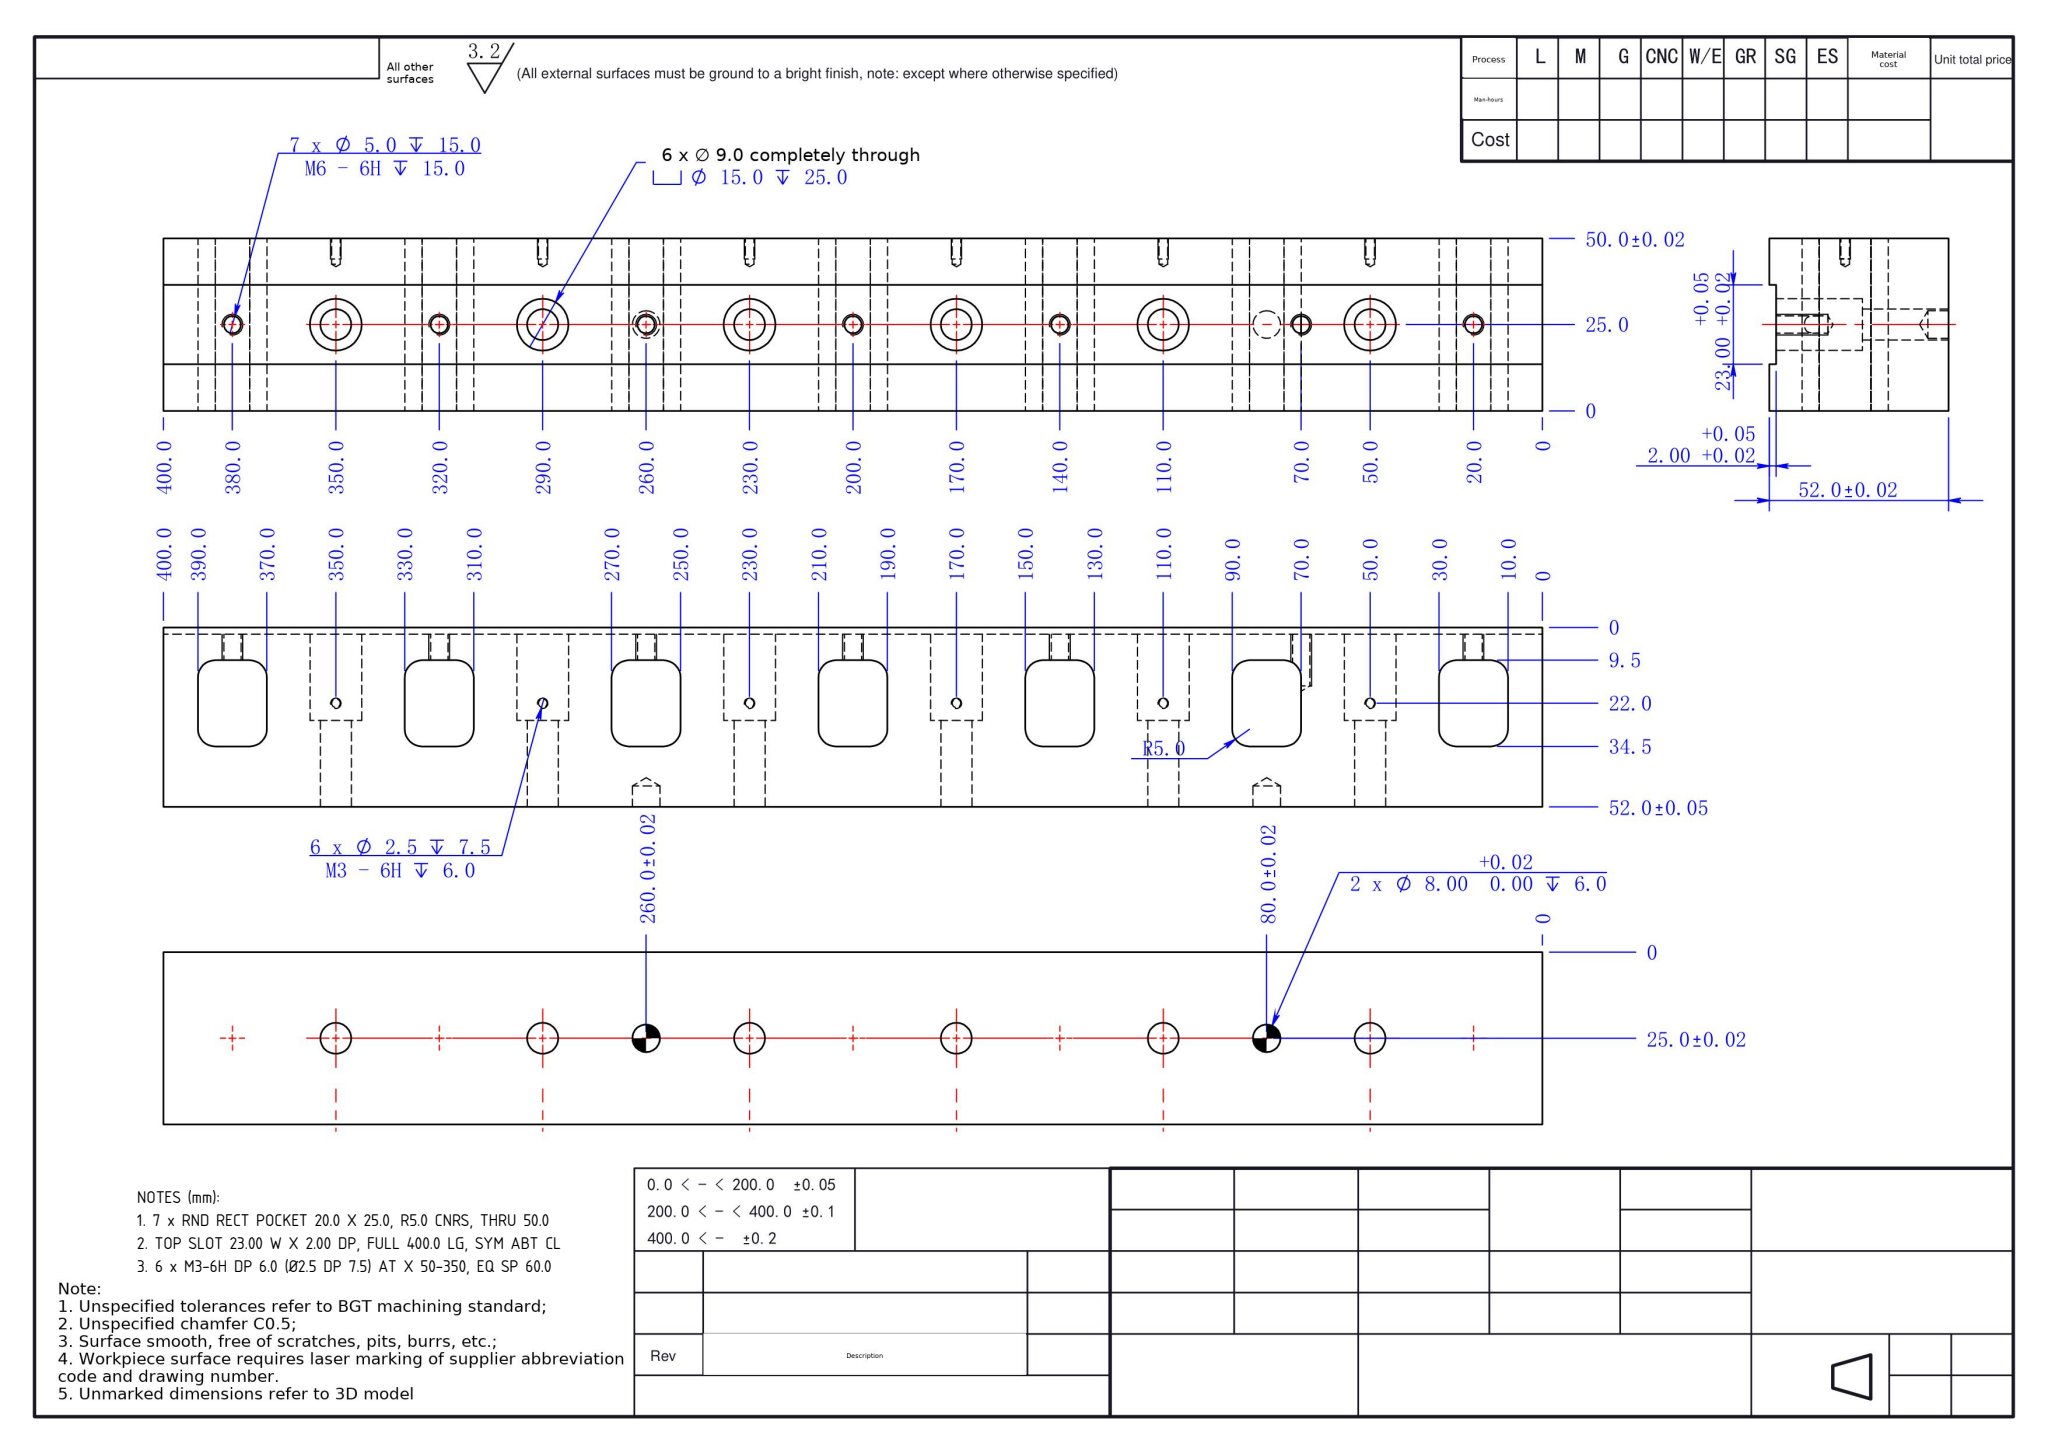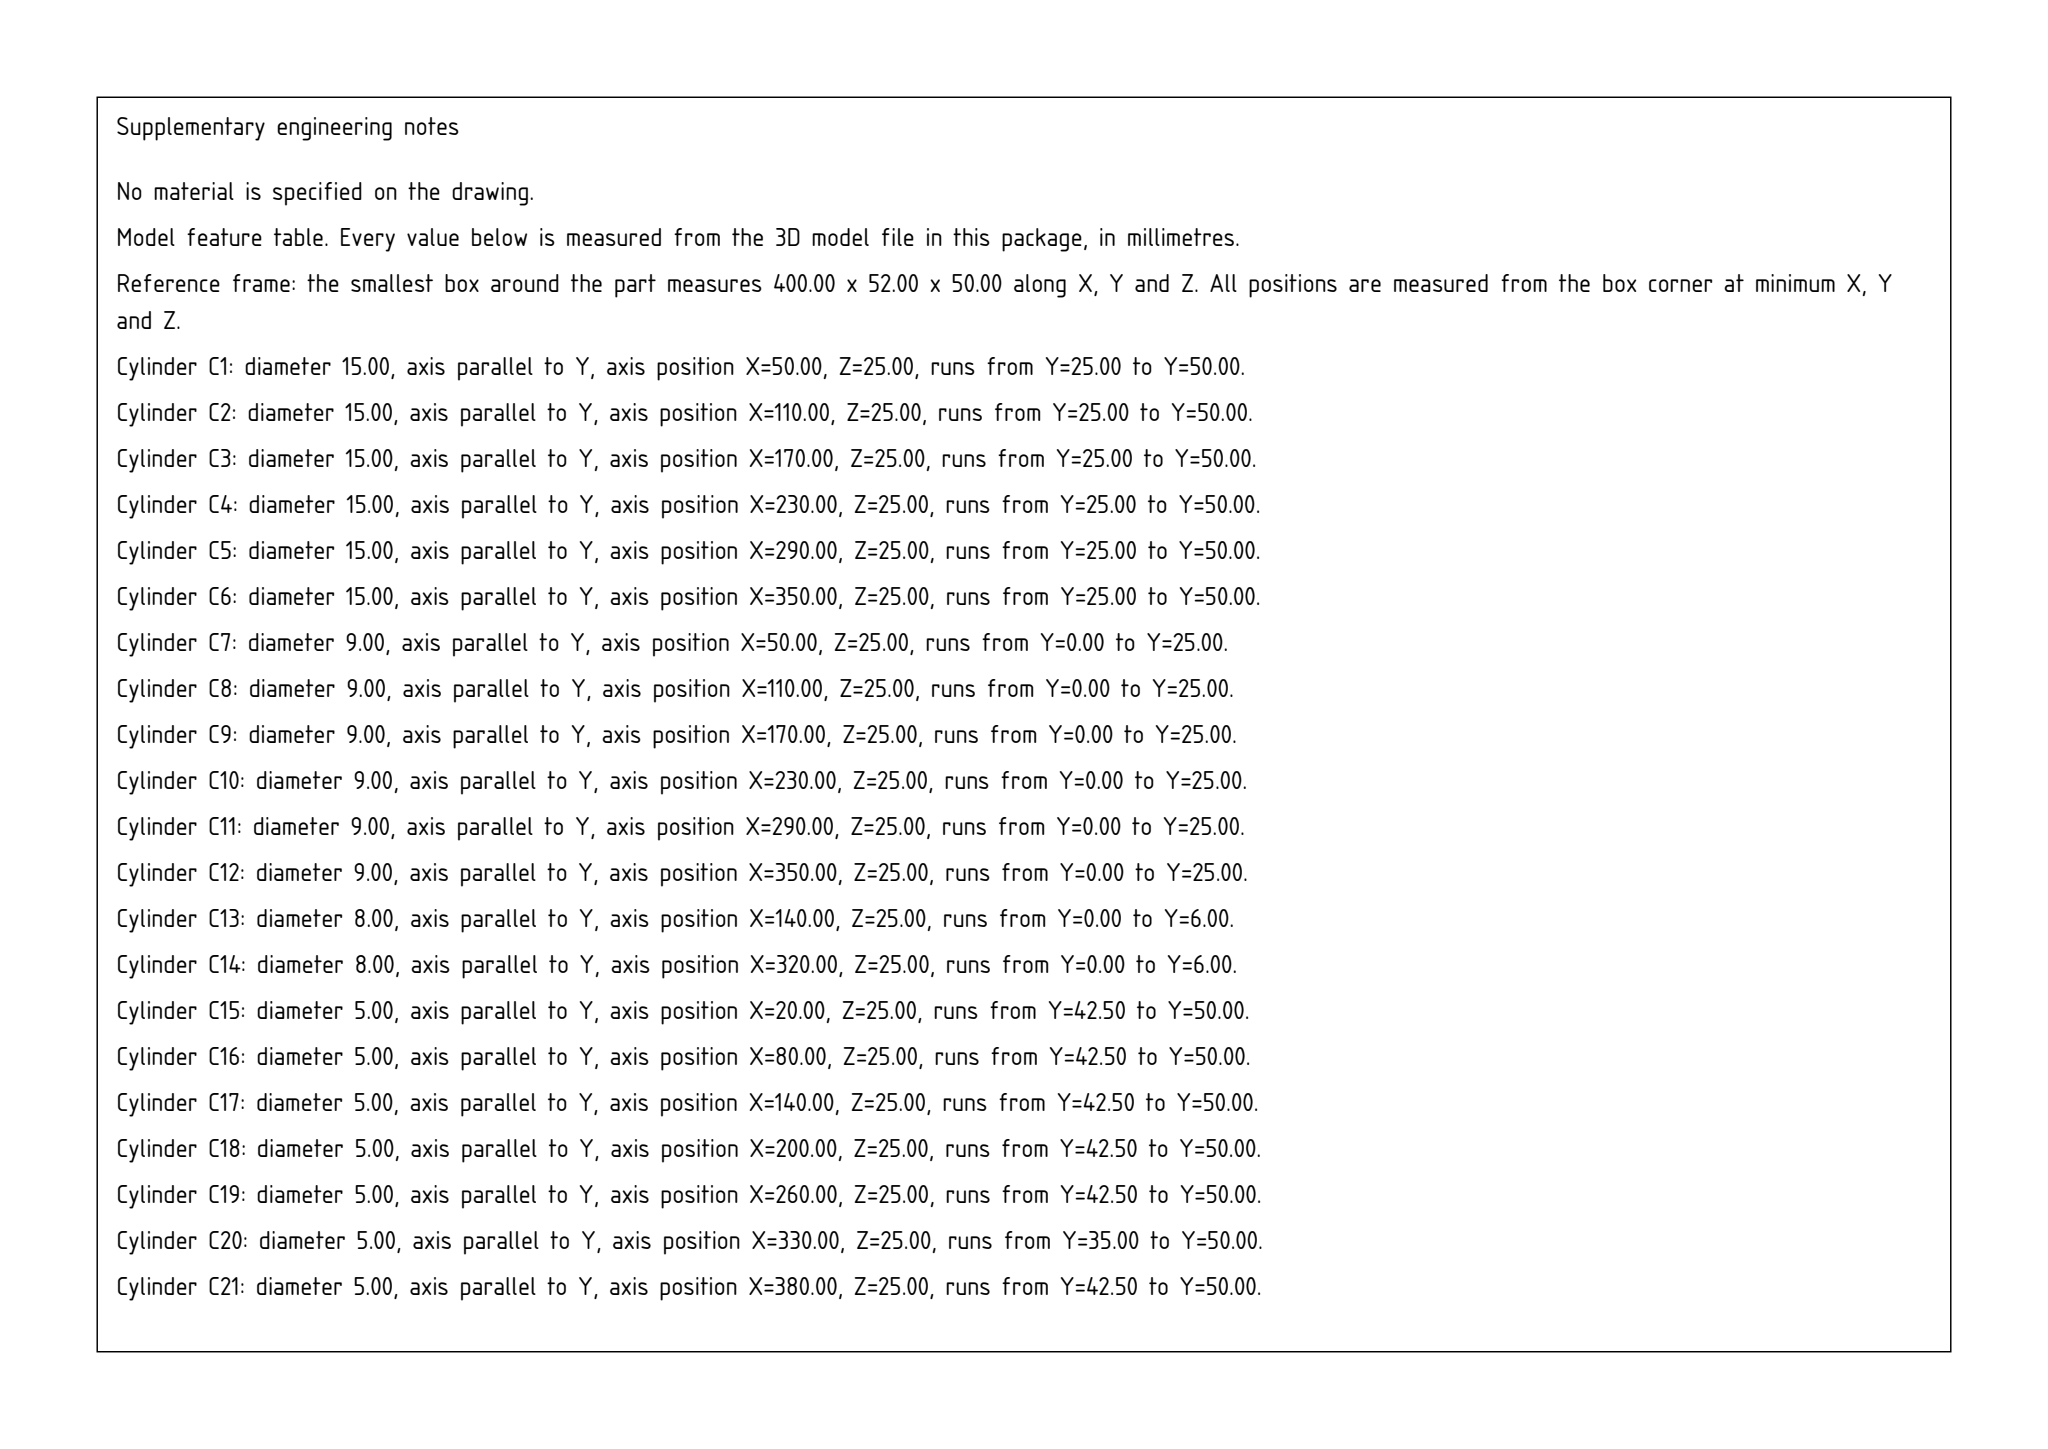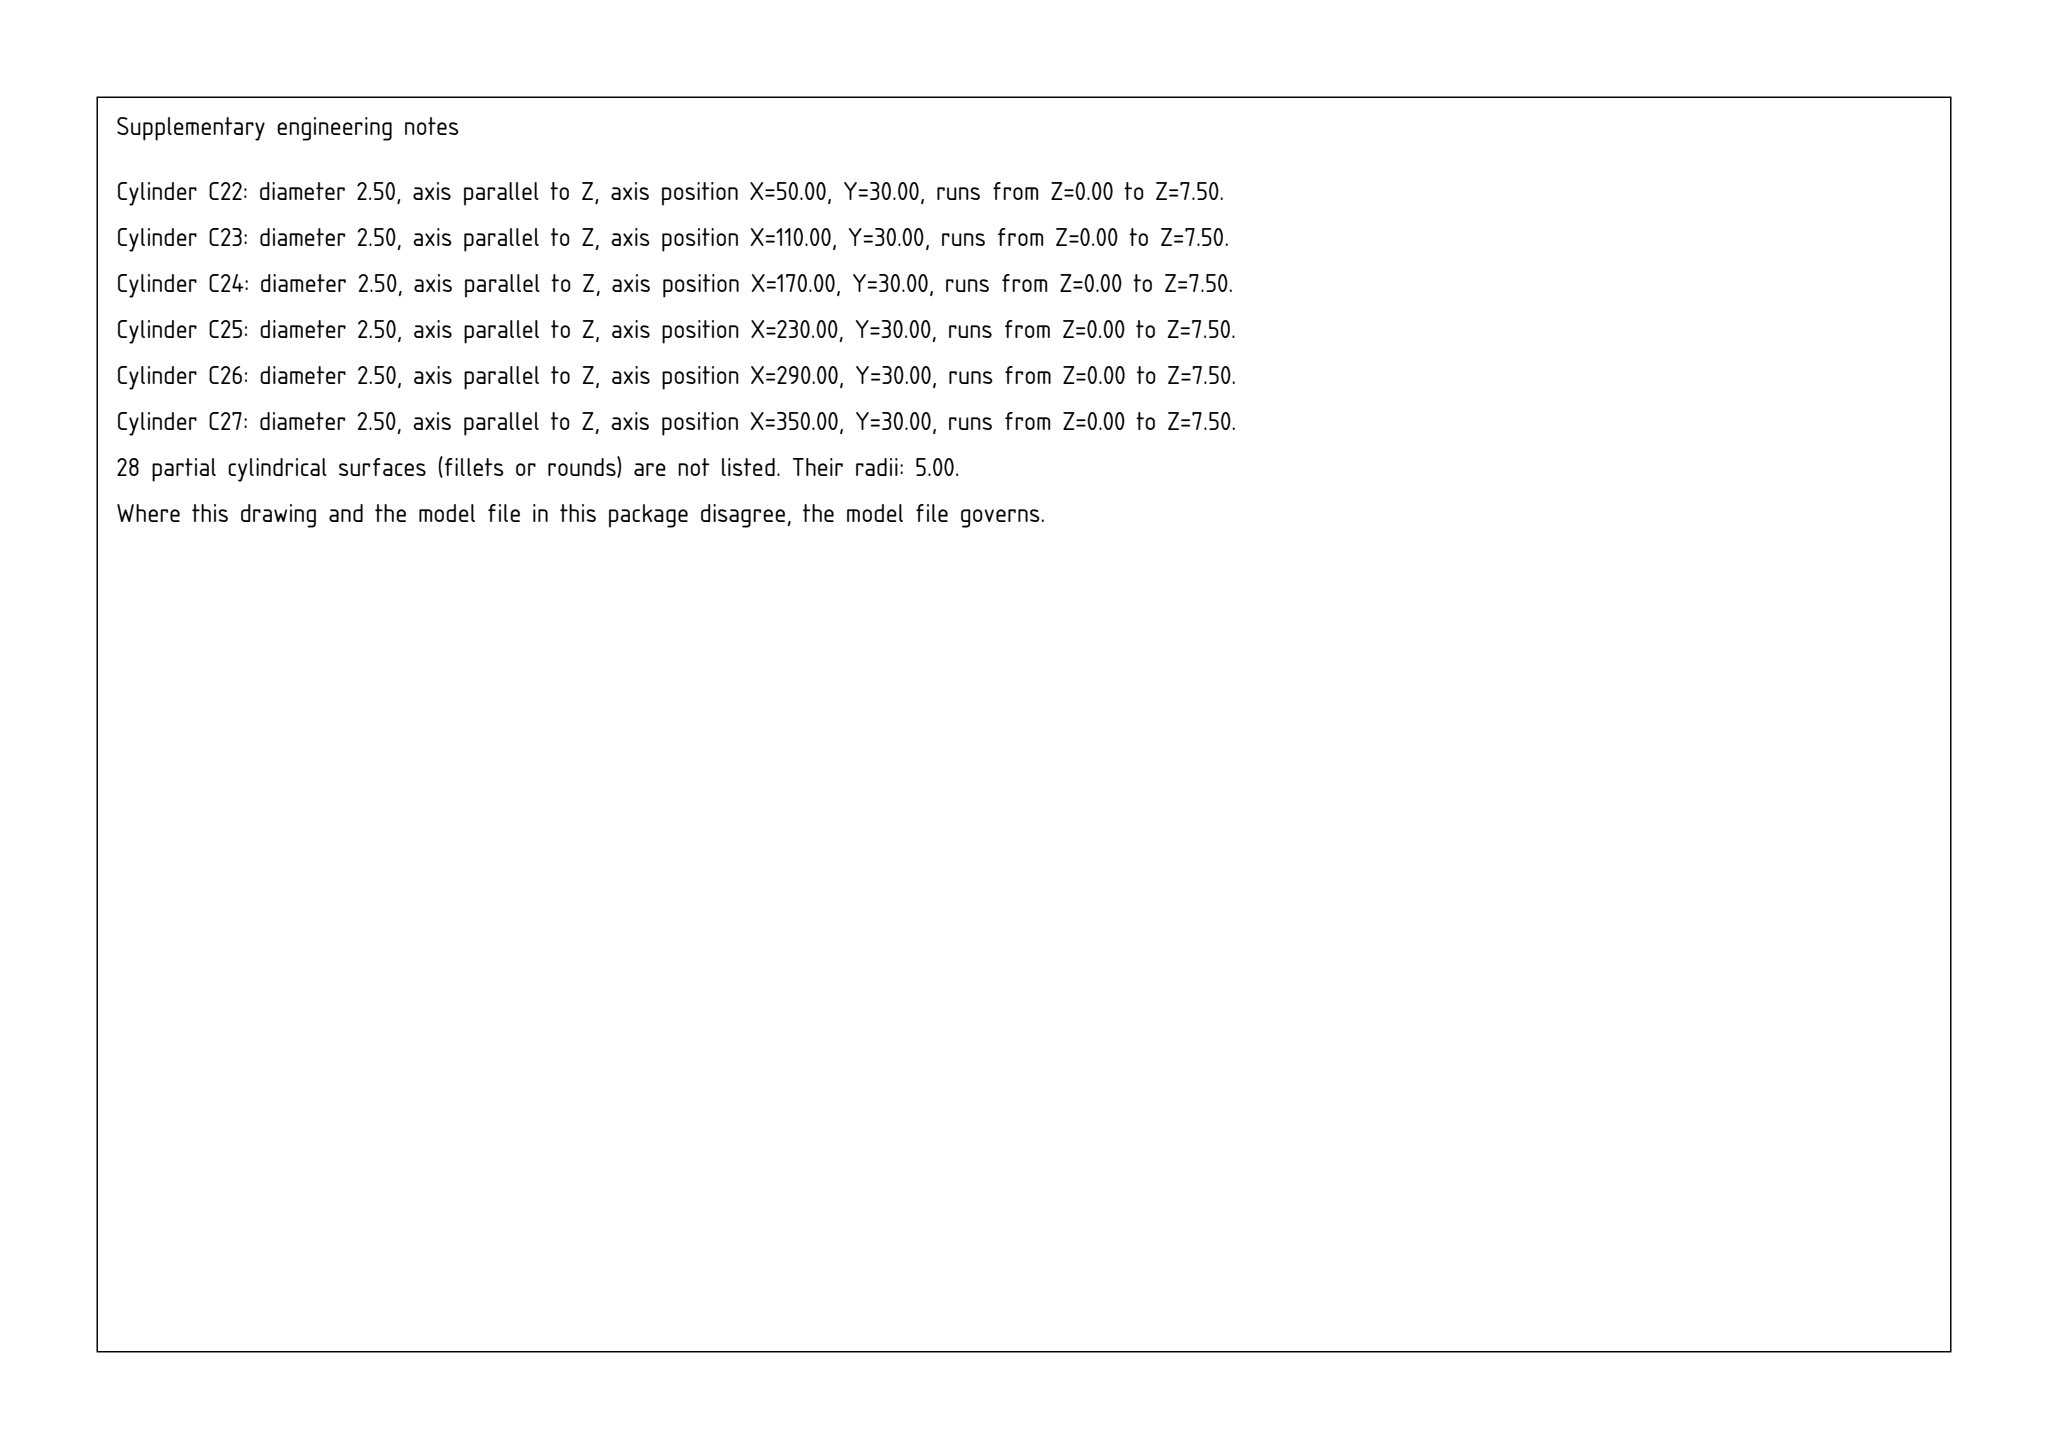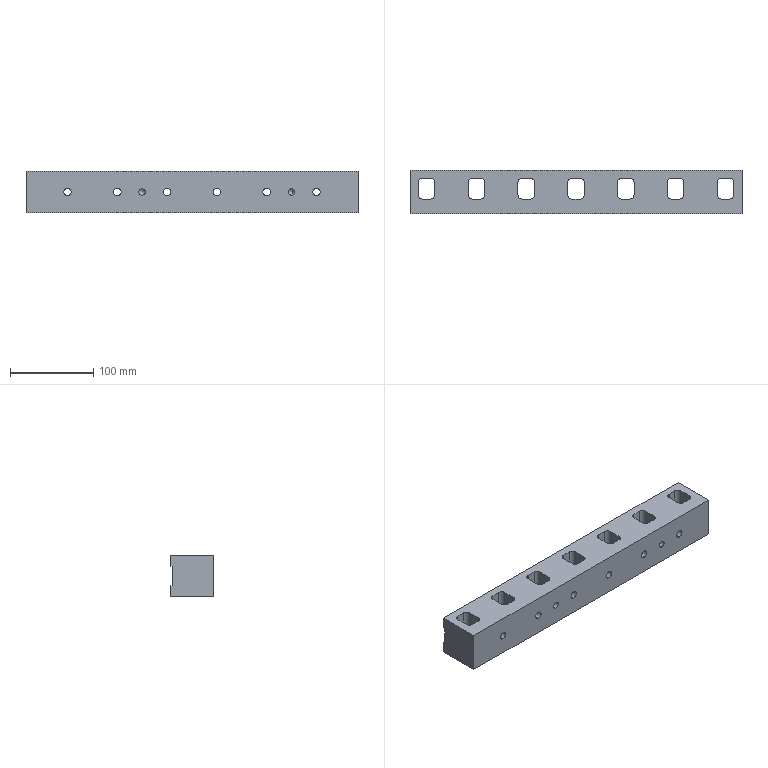Part | SolidWorks | mm | 1 solid | 143 faces | box 400 x 52 x 50 mm | volume 816019 mm3 | cylinder 82 | plane 44 | cone 17 | commonest cylinder face diameters 10 x28 5 x14 2.5 x12 15 x12 9 x12 8 x4
Drawing notes:
7 x RND RECT POCKET 20.0 X 25.0, R5.0 CNRS, THRU 50.0 | from the solid: Ø10 z-axis corner cyls L=50 (full z 0-50) at x=15/25,75/85,...,375/385, y=22.5/37.5; x-planes 10/30...370/390; y-planes 17.5 & 42.5 (7 ea)
TOP SLOT 23.00 W X 2.00 DP, FULL 400.0 LG, SYM ABT CL | from the solid: z-planes 13.5 & 36.5 (23.0 apart, sym about z=25); y-plane 50.0 vs bbox y=52.0 gives 2.0 dp; y=52 face split in 2 => groove runs full 400 length
6 x M3-6H DP 6.0 (Ø2.5 DP 7.5) AT X 50-350, EQ SP 60.0 | from the solid: Ø2.5 z-axis holes at x = 50, 110, 170, 230, 290, 350 (y=30), depth 7.5; 290.0 station missing on drawing